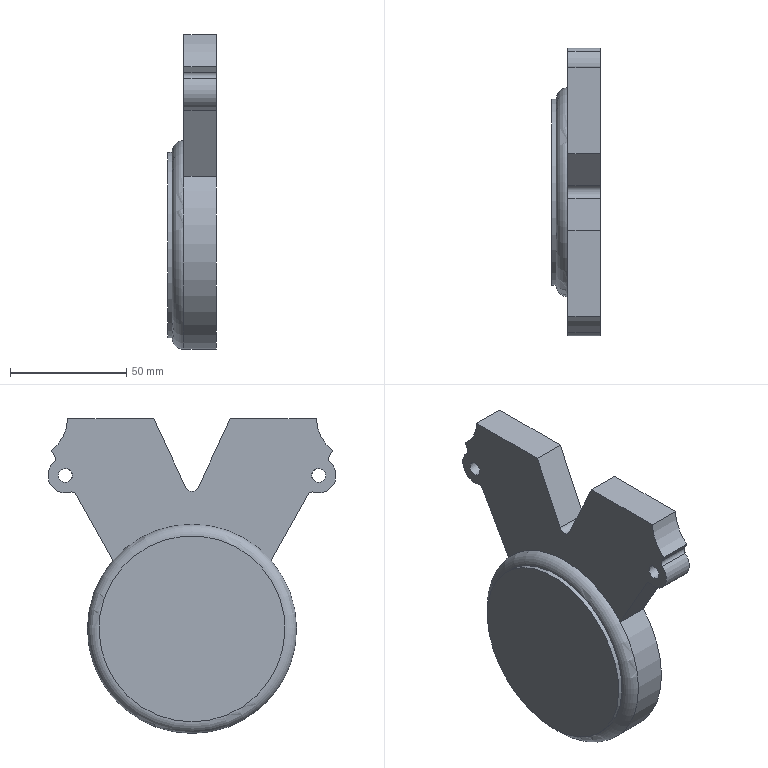Component | NX | FRONT_OUTER_END_CAP | 1 solid | 25 faces | volume 196857 mm3 | cylinder 13 | plane 11 | torus 1 | commonest cylinder face diameters 4 x4 6 x3 15 x2 36 x2 90 x1 80 x1